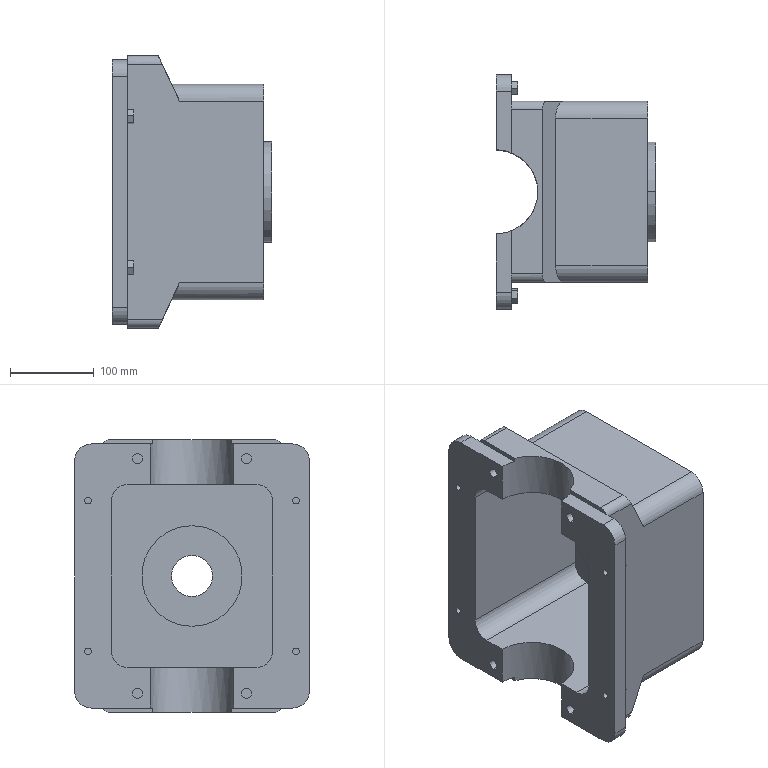Component | SolidWorks | BoxCover-1 | 1 solid | 109 faces | box 190.79 x 280 x 325 mm | volume 4012149 mm3 | plane 67 | cylinder 42 | commonest cylinder face diameters 40 x12 12 x8 8 x8 120 x4 20 x4 49 x2 90 x2 100 x2
build123d program:
from build123d import *

# Parameters (mm, degrees)
BOSS_EXTRUDE1_DEPTH = 18
BOSS_EXTRUDE2_DEPTH = 138
CUT_EXTRUDE1_DEPTH  = 141
CUT_EXTRUDE2_DEPTH  = 336.032
CUT_EXTRUDE3_DEPTH  = 336.032
CUT_EXTRUDE4_DEPTH  = 500
SKETCH7_R           = 4
SKETCH7_R_2         = 6
CUT_EXTRUDE5_DEPTH  = 20
SKETCH8_W           = 429.148
SKETCH8_H           = 306.965
CUT_EXTRUDE6_DEPTH  = 241.959
SKETCH9_W           = 257
SKETCH9_H           = 216
BOSS_EXTRUDE3_DEPTH = 71
BOSS_EXTRUDE4_START = -12
BOSS_EXTRUDE4_DEPTH = 12
FILLET1_R           = 20
FILLET2_R           = 20
FILLET3_R           = 20
FILLET4_R           = 20
SKETCH11_R          = 60
BOSS_EXTRUDE5_DEPTH = 10
SKETCH12_R          = 45
CUT_EXTRUDE7_DEPTH  = 288.07
SKETCH13_R          = 60
SKETCH13_R_2        = 45
BOSS_EXTRUDE6_DEPTH = 38
BOSS_EXTRUDE7_START = -12
SKETCH14_R          = 45
BOSS_EXTRUDE7_DEPTH = 12
SKETCH15_R          = 24.5
CUT_EXTRUDE8_DEPTH  = 252.224
BOSS_EXTRUDE8_DEPTH = 8


with BuildPart() as part:
    # Sketch1 → Boss-Extrude1 (new body)
    with BuildSketch(Plane(origin=(0, 0, 0), x_dir=(0, 0, -1), z_dir=(1, 0, 0))):
        with BuildLine():
            Line((137.5, 140), (-137.5, 140))
            ThreePointArc((-137.5, 140), (-151.642, 134.142), (-157.5, 120))
            Line((-157.5, 120), (-157.5, -120))
            ThreePointArc((-157.5, -120), (-151.642, -134.142), (-137.5, -140))
            Line((-137.5, -140), (137.5, -140))
            ThreePointArc((137.5, -140), (151.642, -134.142), (157.5, -120))
            Line((157.5, -120), (157.5, 120))
            ThreePointArc((157.5, 120), (151.642, 134.142), (137.5, 140))
        make_face()
    extrude(amount=BOSS_EXTRUDE1_DEPTH)

    # Sketch2 → Boss-Extrude2 (add)
    with BuildSketch(Plane(origin=(18, 0, 0), x_dir=(0, 0, -1), z_dir=(1, 0, 0))):
        with BuildLine():
            Line((152.5, 108), (-152.5, 108))
            ThreePointArc((-152.5, 108), (-159.571, 105.071), (-162.5, 98))
            Line((-162.5, 98), (-162.5, -98))
            ThreePointArc((-162.5, -98), (-159.571, -105.071), (-152.5, -108))
            Line((-152.5, -108), (152.5, -108))
            ThreePointArc((152.5, -108), (159.571, -105.071), (162.5, -98))
            Line((162.5, -98), (162.5, 98))
            ThreePointArc((162.5, 98), (159.571, 105.071), (152.5, 108))
        make_face()
    extrude(amount=BOSS_EXTRUDE2_DEPTH)

    # Sketch3 → Cut-Extrude1 (cut)
    with BuildSketch(Plane.ZY):
        with BuildLine():
            Line((89.5, 96), (-89.5, 96))
            ThreePointArc((-89.5, 96), (-103.642, 90.142), (-109.5, 76))
            Line((-109.5, 76), (-109.5, -76))
            ThreePointArc((-109.5, -76), (-103.642, -90.142), (-89.5, -96))
            Line((-89.5, -96), (89.5, -96))
            ThreePointArc((89.5, -96), (103.642, -90.142), (109.5, -76))
            Line((109.5, -76), (109.5, 76))
            ThreePointArc((109.5, 76), (103.642, 90.142), (89.5, 96))
        make_face()
    extrude(amount=-CUT_EXTRUDE1_DEPTH, mode=Mode.SUBTRACT)

    # Sketch4 → Cut-Extrude2 (cut, through all)
    with BuildSketch(Plane.XZ.offset(108)):
        Polygon((156, 0), (156, 105), (151, 105), (151, -105), (156, -105), align=None)
    extrude(amount=-CUT_EXTRUDE2_DEPTH, mode=Mode.SUBTRACT)

    # Sketch5 → Cut-Extrude3 (cut, through all)
    with BuildSketch(Plane.XZ.offset(108)):
        Polygon((71.095, -128.5), (109.795, -128.5), (109.795, -162.5), (55.218, -162.5), align=None)
        Polygon((55.218, 162.5), (71.095, 128.5), (109.795, 128.5), (109.795, 162.5), align=None)
    extrude(amount=-CUT_EXTRUDE3_DEPTH, mode=Mode.SUBTRACT)

    # Sketch6 → Cut-Extrude4 (cut, symmetric)
    with BuildSketch(Plane(origin=(0, 0, -157.5), x_dir=(-1, 0, 0), z_dir=(0, 0, -1))):
        with BuildLine():
            Line((0, 50), (0, -50))
            ThreePointArc((0, -50), (-50, 0), (0, 50))
        make_face()
    extrude(amount=CUT_EXTRUDE4_DEPTH, both=True, mode=Mode.SUBTRACT)

    # Sketch7 → Cut-Extrude5 (cut)
    with BuildSketch(Plane.ZY):
        with Locations((-90, 124)):
            Circle(SKETCH7_R)
        with Locations((140, -65)):
            Circle(SKETCH7_R_2)
        with Locations(Location((90, 124, 0), (0, 0, 180))):
            Circle(SKETCH7_R)
        with Locations((90, -124)):
            Circle(SKETCH7_R)
        with Locations(Location((-90, -124, 0), (0, 0, 180))):
            Circle(SKETCH7_R)
        with Locations(Location((140, 65, 0), (0, 0, 180))):
            Circle(SKETCH7_R_2)
        with Locations((-140, 65)):
            Circle(SKETCH7_R_2)
        with Locations(Location((-140, -65, 0), (0, 0, 180))):
            Circle(SKETCH7_R_2)
    extrude(amount=-CUT_EXTRUDE5_DEPTH, mode=Mode.SUBTRACT)

    # Sketch8 → Cut-Extrude6 (cut, through all)
    with BuildSketch(Plane.ZY.offset(-109.795)):
        Rectangle(SKETCH8_W, SKETCH8_H)
    extrude(amount=-CUT_EXTRUDE6_DEPTH, mode=Mode.SUBTRACT)

    # Sketch9 → Boss-Extrude3 (add)
    with BuildSketch(Plane(origin=(109.795, 0, 0), x_dir=(0, 0, -1), z_dir=(1, 0, 0))):
        Rectangle(SKETCH9_W, SKETCH9_H)
        with BuildLine():
            Line((-89.5, 96), (89.5, 96))
            ThreePointArc((89.5, 96), (103.642, 90.142), (109.5, 76))
            Line((109.5, 76), (109.5, -76))
            ThreePointArc((109.5, -76), (103.642, -90.142), (89.5, -96))
            Line((89.5, -96), (-89.5, -96))
            ThreePointArc((-89.5, -96), (-103.642, -90.142), (-109.5, -76))
            Line((-109.5, -76), (-109.5, 76))
            ThreePointArc((-109.5, 76), (-103.642, 90.142), (-89.5, 96))
        make_face(mode=Mode.SUBTRACT)
    extrude(amount=BOSS_EXTRUDE3_DEPTH)

    # Sketch10 → Boss-Extrude4 (add)
    with BuildSketch(Plane(origin=(180.795, 0, 0), x_dir=(0, 0, -1), z_dir=(1, 0, 0)).offset(BOSS_EXTRUDE4_START)):
        with BuildLine():
            Line((89.5, 96), (-89.5, 96))
            ThreePointArc((-89.5, 96), (-103.642, 90.142), (-109.5, 76))
            Line((-109.5, 76), (-109.5, -76))
            ThreePointArc((-109.5, -76), (-103.642, -90.142), (-89.5, -96))
            Line((-89.5, -96), (89.5, -96))
            ThreePointArc((89.5, -96), (103.642, -90.142), (109.5, -76))
            Line((109.5, -76), (109.5, 76))
            ThreePointArc((109.5, 76), (103.642, 90.142), (89.5, 96))
        make_face()
    extrude(amount=BOSS_EXTRUDE4_DEPTH)

    # Fillet1
    fillet1_edges = [part.edges().sort_by_distance(p)[0] for p in [
        (125.945, -108, 128.5),
    ]]
    fillet(fillet1_edges, radius=FILLET1_R)

    # Fillet2
    fillet2_edges = [part.edges().sort_by_distance(p)[0] for p in [
        (125.945, -108, -128.5),
    ]]
    fillet(fillet2_edges, radius=FILLET2_R)

    # Fillet3
    fillet3_edges = [part.edges().sort_by_distance(p)[0] for p in [
        (125.945, 108, -128.5),
    ]]
    fillet(fillet3_edges, radius=FILLET3_R)

    # Fillet4
    fillet4_edges = [part.edges().sort_by_distance(p)[0] for p in [
        (125.945, 108, 128.5),
    ]]
    fillet(fillet4_edges, radius=FILLET4_R)

    # Sketch11 → Boss-Extrude5 (add)
    with BuildSketch(Plane(origin=(180.795, 0, 0), x_dir=(0, 0, -1), z_dir=(1, 0, 0))):
        with Locations(Location((0, 0, 0), (0, 0, 180))):
            Circle(SKETCH11_R)
    extrude(amount=BOSS_EXTRUDE5_DEPTH)

    # Sketch12 → Cut-Extrude7 (cut, through all)
    with BuildSketch(Plane(origin=(190.795, 0, 0), x_dir=(0, 0, -1), z_dir=(1, 0, 0))):
        Circle(SKETCH12_R)
    extrude(amount=-CUT_EXTRUDE7_DEPTH, mode=Mode.SUBTRACT)

    # Sketch13 → Boss-Extrude6 (add)
    with BuildSketch(Plane.ZY.offset(-168.795)):
        Circle(SKETCH13_R)
        with Locations(Location((0, 0, 0), (0, 0, 180))):
            Circle(SKETCH13_R_2, mode=Mode.SUBTRACT)
    extrude(amount=BOSS_EXTRUDE6_DEPTH)

    # Sketch14 → Boss-Extrude7 (add)
    with BuildSketch(Plane.ZY.offset(-130.795).offset(BOSS_EXTRUDE7_START)):
        with Locations(Location((0, 0, 0), (0, 0, 180))):
            Circle(SKETCH14_R)
    extrude(amount=BOSS_EXTRUDE7_DEPTH)

    # Sketch15 → Cut-Extrude8 (cut, through all)
    with BuildSketch(Plane.ZY.offset(-130.795)):
        Circle(SKETCH15_R)
    extrude(amount=-CUT_EXTRUDE8_DEPTH, mode=Mode.SUBTRACT)

    # Sketch16 → Boss-Extrude8 (add)
    with BuildSketch(Plane(origin=(18, 0, 0), x_dir=(0, 0, -1), z_dir=(1, 0, 0))):
        Polygon((-94, 116.008), (-85.078, 116.54), (-81.078, 124.532), (-86, 131.992), (-94.922, 131.46), (-98.922, 123.468), align=None)
        Polygon((86, 116.54), (94.461, 116.806), (98.461, 124.266), (94, 131.46), (85.539, 131.194), (81.539, 123.734), align=None)
        Polygon((-91.518, -133.066), (-82.908, -129.848), (-81.39, -120.782), (-88.482, -114.934), (-97.092, -118.152), (-98.61, -127.218), align=None)
        Polygon((90, -133.066), (97.851, -128.533), (97.851, -119.467), (90, -114.934), (82.149, -119.467), (82.149, -128.533), align=None)
    extrude(amount=BOSS_EXTRUDE8_DEPTH)


solid = part.part

# Placed as in the assembly
solid = solid.moved(Location((35.733, 15.31, -110), (0, 0, 0)))